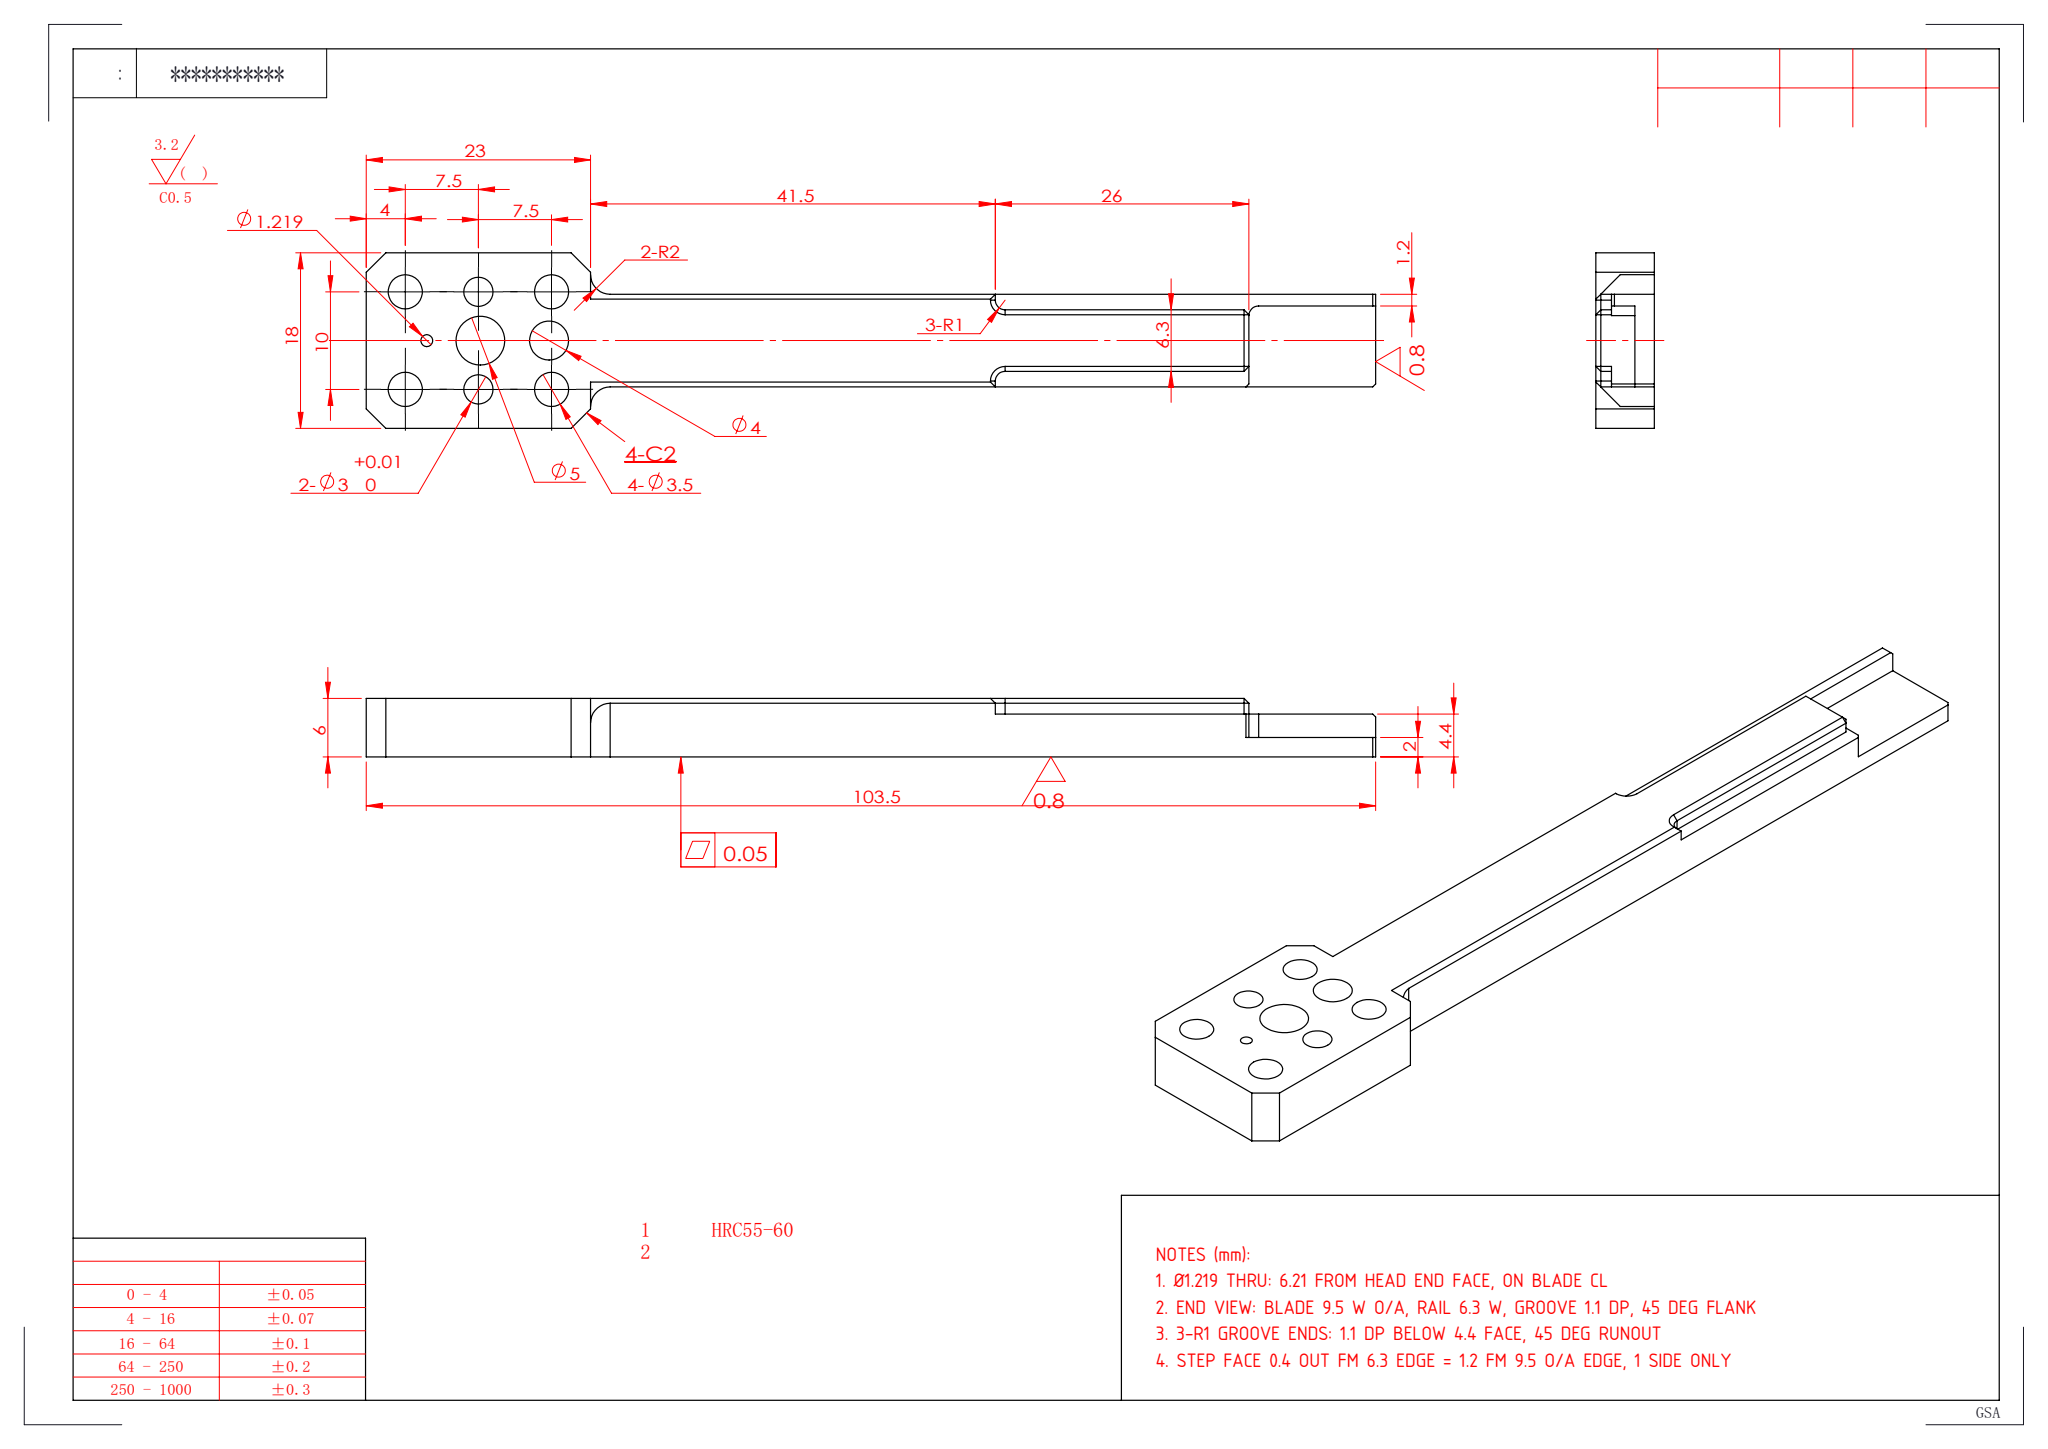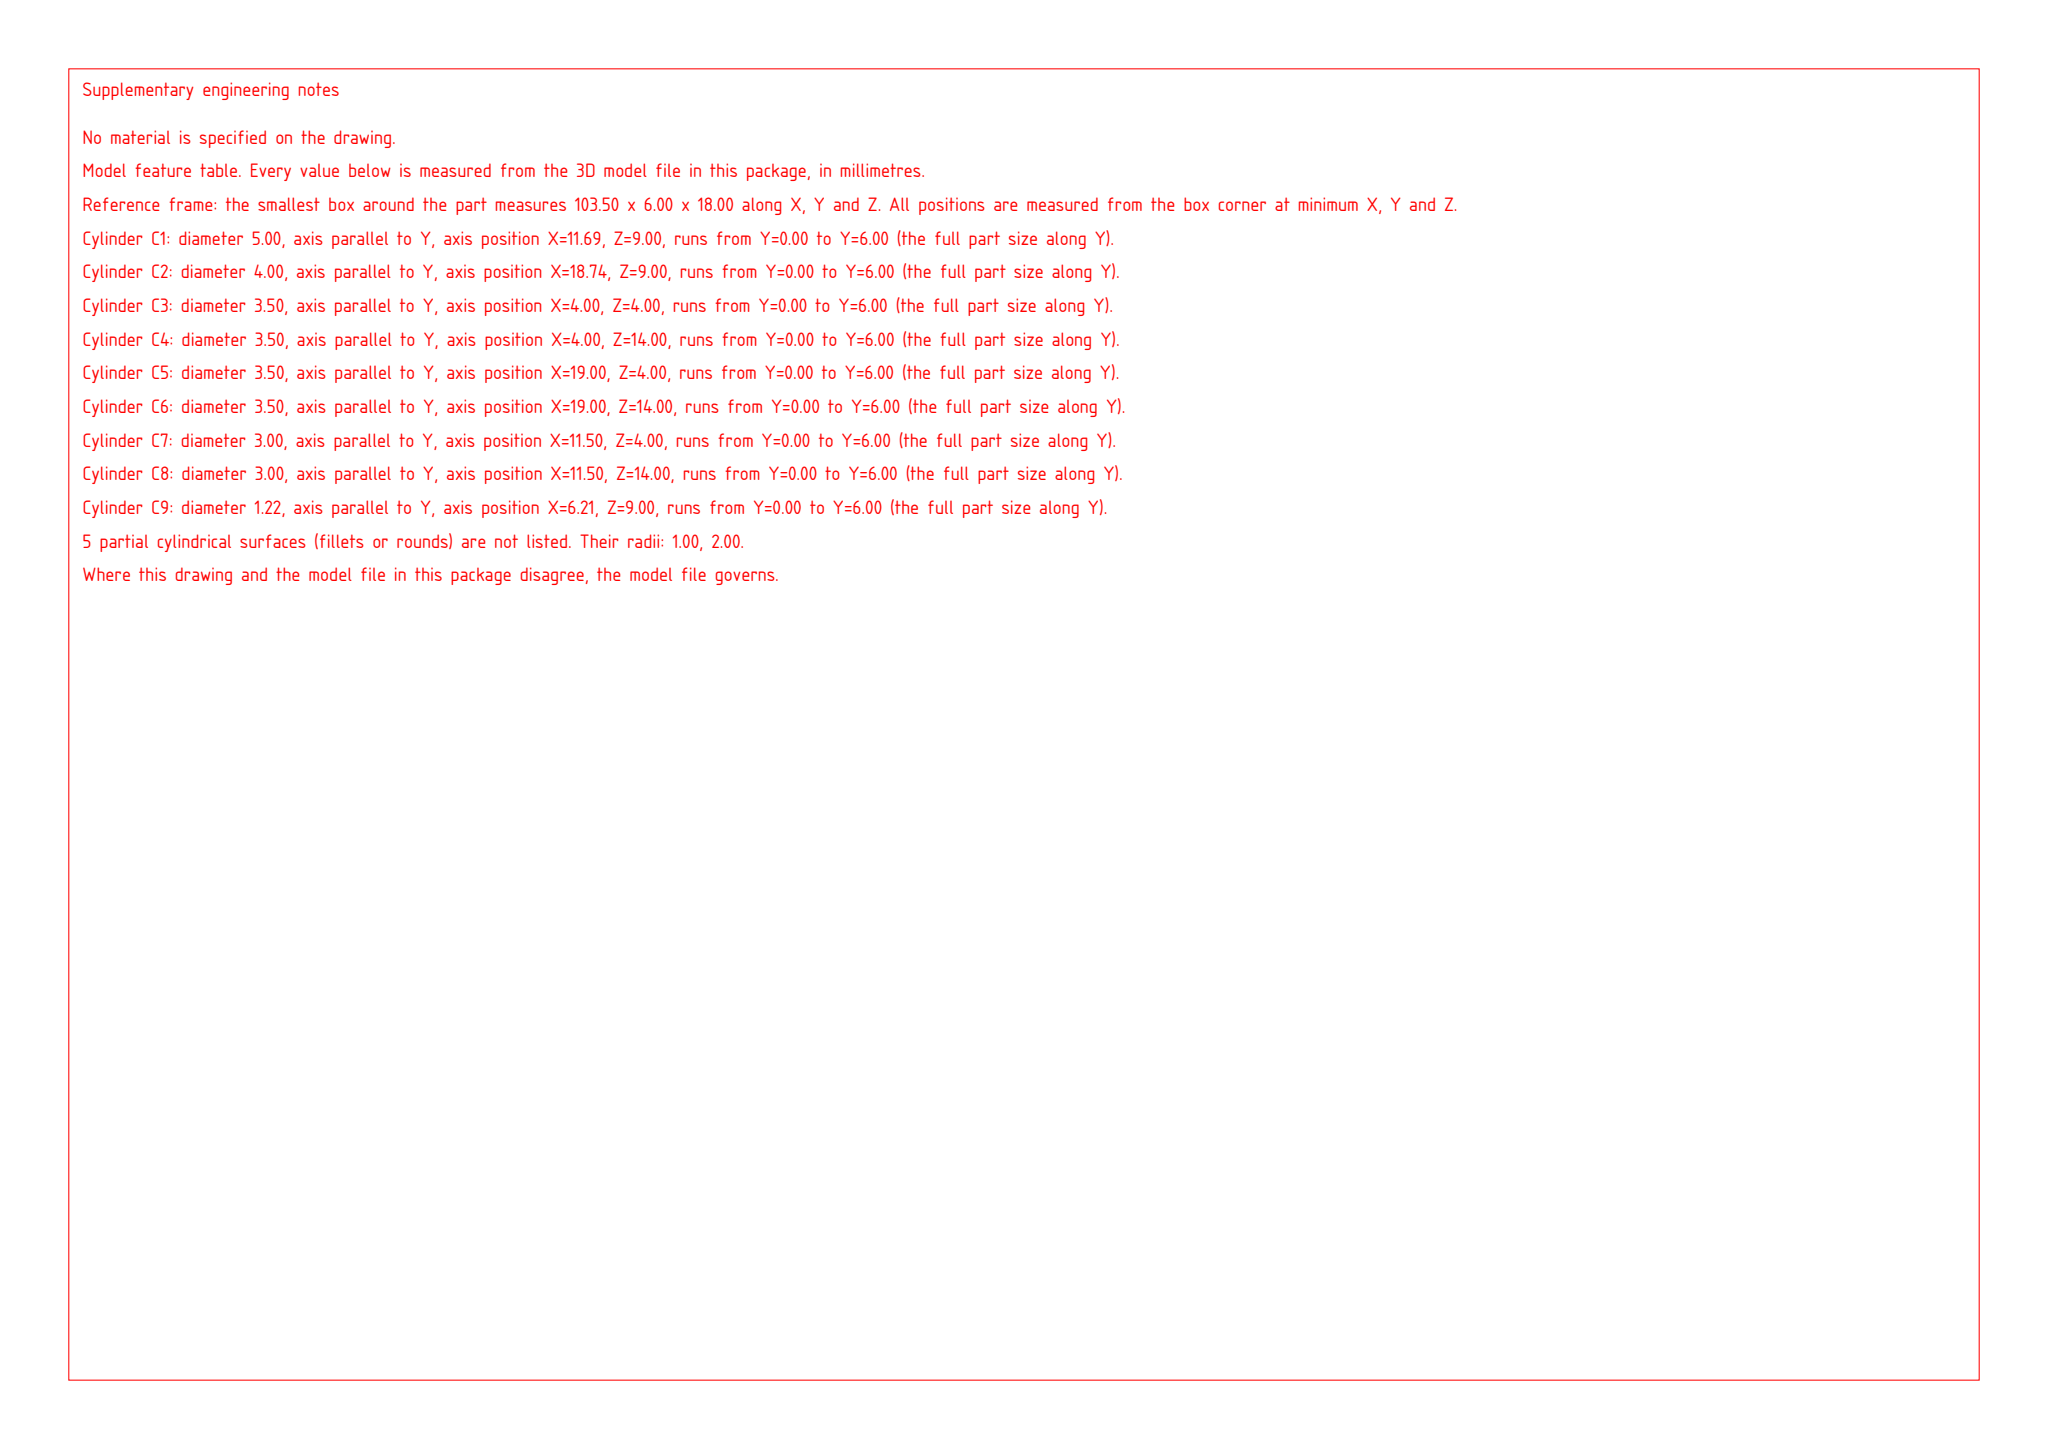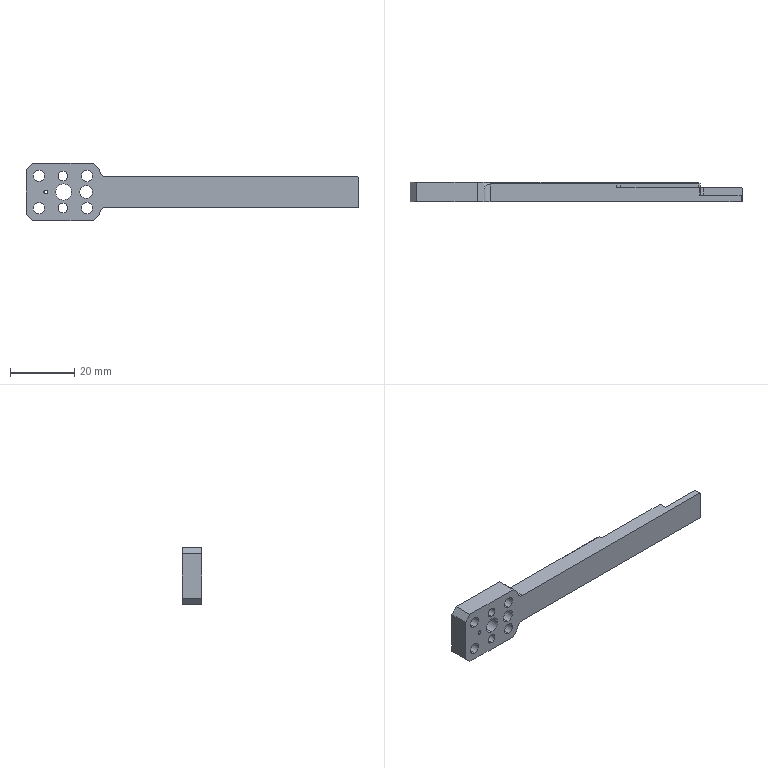Part | SolidWorks | mm | 1 solid | 62 faces | box 103.5 x 6 x 18 mm | volume 5910 mm3 | plane 37 | cylinder 23 | cone 2 | commonest cylinder face diameters 3.5 x8 4 x4 3 x4 2 x3 1.219 x2 5 x2
Drawing notes:
Ø1.219 THRU: 6.21 FROM HEAD END FACE, ON BLADE CL | from the solid: cyl dia 1.219, axis y, pos x=6.21 z=9.0, len 6.0 (thru 6 thk); head end face = plane x=0; blade CL z=9.0 of 18 wide head
END VIEW: BLADE 9.5 W O/A, RAIL 6.3 W, GROOVE 1.1 DP, 45 DEG FLANK | from the solid: z planes 4.25 & 13.75 (9.5 o/a), 5.85 & 12.15 (6.3 rail); Ø2 cyl len 1.1 = groove depth; cone incl angle 90 deg (45 deg per flank), ref dia 2.0
3-R1 GROOVE ENDS: 1.1 DP BELOW 4.4 FACE, 45 DEG RUNOUT | from the solid: Ø2 cyls at x=65.5 (z=4.85, 13.15) len 1.1 in y; y planes 2 / 4.4 / 6; 90 deg cone ref dia 2 at groove ends
STEP FACE 0.4 OUT FM 6.3 EDGE = 1.2 FM 9.5 O/A EDGE, 1 SIDE ONLY | from the solid: z planes 4.25, 5.45, 5.85 (count 1 each); 5.85-5.45=0.4, 5.45-4.25=1.2; no matching plane at 13.55 on opposite side
build123d program:
from build123d import *

# Parameters (mm, degrees)
BOSS_EXTRUDE1_DEPTH = 9
SKETCH2_W           = 80.5
SKETCH2_H           = 4.25
CUT_EXTRUDE1_DEPTH  = 104.968
CHAMFER1_SIZE       = 2
CHAMFER4_SIZE       = 2
BOSS_EXTRUDE3_DEPTH = 4
SKETCH9_W           = 13
SKETCH9_H           = 1.2
CUT_EXTRUDE3_DEPTH  = 1.6
FILLET1_R           = 1
CUT_EXTRUDE4_DEPTH  = 1.6
CHAMFER10_SIZE      = 0.5
CHAMFER11_SIZE      = 0.3
SKETCH11_R          = 1.75
CUT_EXTRUDE5_DEPTH  = 105.064
SKETCH12_R          = 1.5
CUT_EXTRUDE6_DEPTH  = 105.064
FILLET2_R           = 2
SKETCH13_R          = 0.6097
SKETCH13_R_2        = 2.5
SKETCH13_R_3        = 2
CUT_EXTRUDE7_DEPTH  = 10


with BuildPart() as part:
    # Sketch1 → Boss-Extrude1 (new, symmetric)
    with BuildSketch(Plane.XY):
        Polygon((23, 6), (23, 2), (103.5, 2), (103.5, 0), (0, 0), (0, 6), align=None)
    extrude(amount=BOSS_EXTRUDE1_DEPTH, both=True)

    # Sketch2 → Cut-Extrude1 (cut, through all)
    with BuildSketch(Plane(origin=(0, 2, 0), x_dir=(1, 0, 0), z_dir=(0, 1, 0))):
        with Locations((63.25, 6.875)):
            Rectangle(SKETCH2_W, SKETCH2_H)
        with Locations((63.25, -6.875)):
            Rectangle(SKETCH2_W, SKETCH2_H)
    extrude(amount=-CUT_EXTRUDE1_DEPTH, mode=Mode.SUBTRACT)

    # Chamfer1
    chamfer1_edges = [part.edges().sort_by_distance(p)[0] for p in [
        (23, 3, 9),
        (23, 3, -9),
    ]]
    chamfer(chamfer1_edges, length=CHAMFER1_SIZE)

    # Chamfer4
    chamfer4_edges = [part.edges().sort_by_distance(p)[0] for p in [
        (0, 3, 9),
        (0, 3, -9),
    ]]
    chamfer(chamfer4_edges, length=CHAMFER4_SIZE)

    # Sketch8 → Boss-Extrude3 (add)
    with BuildSketch(Plane(origin=(0, 2, 0), x_dir=(1, 0, 0), z_dir=(0, 1, 0))):
        Polygon((23, 4.75), (103.5, 4.75), (103.5, 3.55), (90.5, 3.55), (90.5, -4.75), (23, -4.75), align=None)
    extrude(amount=BOSS_EXTRUDE3_DEPTH)

    # Sketch9 → Cut-Extrude3 (cut)
    with BuildSketch(Plane(origin=(0, 6, 0), x_dir=(1, 0, 0), z_dir=(0, 1, 0))):
        with Locations((97, 4.15)):
            Rectangle(SKETCH9_W, SKETCH9_H)
    extrude(amount=-CUT_EXTRUDE3_DEPTH, mode=Mode.SUBTRACT)

    # Fillet1
    fillet1_edges = [part.edges().sort_by_distance(p)[0] for p in [
        (90.5, 3.2, -3.55),
    ]]
    fillet(fillet1_edges, radius=FILLET1_R)

    # Sketch10 → Cut-Extrude4 (cut)
    with BuildSketch(Plane(origin=(0, 6, 0), x_dir=(1, 0, 0), z_dir=(0, 1, 0))):
        with BuildLine():
            Line((90.5, 4.75), (64.5, 4.75))
            Line((64.5, 4.75), (64.5, 4.15))
            ThreePointArc((64.5, 4.15), (64.793, 3.443), (65.5, 3.15))
            Line((65.5, 3.15), (90.5, 3.15))
            Line((90.5, 3.15), (90.5, 4.75))
        make_face()
        with BuildLine():
            Line((64.5, -4.75), (64.5, -4.15))
            ThreePointArc((64.5, -4.15), (64.793, -3.443), (65.5, -3.15))
            Line((65.5, -3.15), (90.5, -3.15))
            Line((90.5, -3.15), (90.5, -4.75))
            Line((90.5, -4.75), (64.5, -4.75))
        make_face()
    extrude(amount=-CUT_EXTRUDE4_DEPTH, mode=Mode.SUBTRACT)

    # Chamfer10
    chamfer10_edges = [part.edges().sort_by_distance(p)[0] for p in [
        (90.5, 6, 0),
        (64.5, 6, -4.45),
        (64.793, 6, -3.443),
        (78, 6, -3.15),
        (90.5, 5.2, -3.15),
        (43.75, 6, 4.75),
        (64.793, 6, 3.443),
        (64.5, 6, 4.45),
        (78, 6, 3.15),
        (90.5, 5.2, 3.15),
        (43.75, 6, -4.75),
    ]]
    chamfer(chamfer10_edges, length=CHAMFER10_SIZE)

    # Chamfer11
    chamfer11_edges = [part.edges().sort_by_distance(p)[0] for p in [
        (90.5, 3.2, 4.75),
        (103.5, 1, 4.75),
        (103.5, 4.4, -4.15),
    ]]
    chamfer(chamfer11_edges, length=CHAMFER11_SIZE)

    # Sketch11 → Cut-Extrude5 (cut, through all)
    with BuildSketch(Plane(origin=(0, 6, 0), x_dir=(1, 0, 0), z_dir=(0, 1, 0))):
        with Locations(Location((4, 5, 0), (0, 0, 270))):
            Circle(SKETCH11_R)
        with Locations(Location((19, 5, 0), (0, 0, 270))):
            Circle(SKETCH11_R)
        with Locations(Location((19, -5, 0), (0, 0, 90))):
            Circle(SKETCH11_R)
        with Locations(Location((4, -5, 0), (0, 0, 90))):
            Circle(SKETCH11_R)
    extrude(amount=-CUT_EXTRUDE5_DEPTH, mode=Mode.SUBTRACT)

    # Sketch12 → Cut-Extrude6 (cut, through all)
    with BuildSketch(Plane(origin=(0, 6, 0), x_dir=(1, 0, 0), z_dir=(0, 1, 0))):
        with Locations(Location((11.5, 5, 0), (0, 0, 270))):
            Circle(SKETCH12_R)
        with Locations(Location((11.5, -5, 0), (0, 0, 270))):
            Circle(SKETCH12_R)
    extrude(amount=-CUT_EXTRUDE6_DEPTH, mode=Mode.SUBTRACT)

    # Fillet2
    fillet2_edges = [part.edges().sort_by_distance(p)[0] for p in [
        (23, 2.75, -4.75),
        (23, 2.75, 4.75),
    ]]
    fillet(fillet2_edges, radius=FILLET2_R)

    # Sketch13 → Cut-Extrude7 (cut)
    with BuildSketch(Plane(origin=(0, 6, 0), x_dir=(1, 0, 0), z_dir=(0, 1, 0))):
        with Locations(Location((6.208, 0, 0), (0, 0, 270))):
            Circle(SKETCH13_R)
        with Locations(Location((11.695, 0, 0), (0, 0, 270))):
            Circle(SKETCH13_R_2)
        with Locations(Location((18.741, 0, 0), (0, 0, 270))):
            Circle(SKETCH13_R_3)
    extrude(amount=-CUT_EXTRUDE7_DEPTH, mode=Mode.SUBTRACT)


solid = part.part